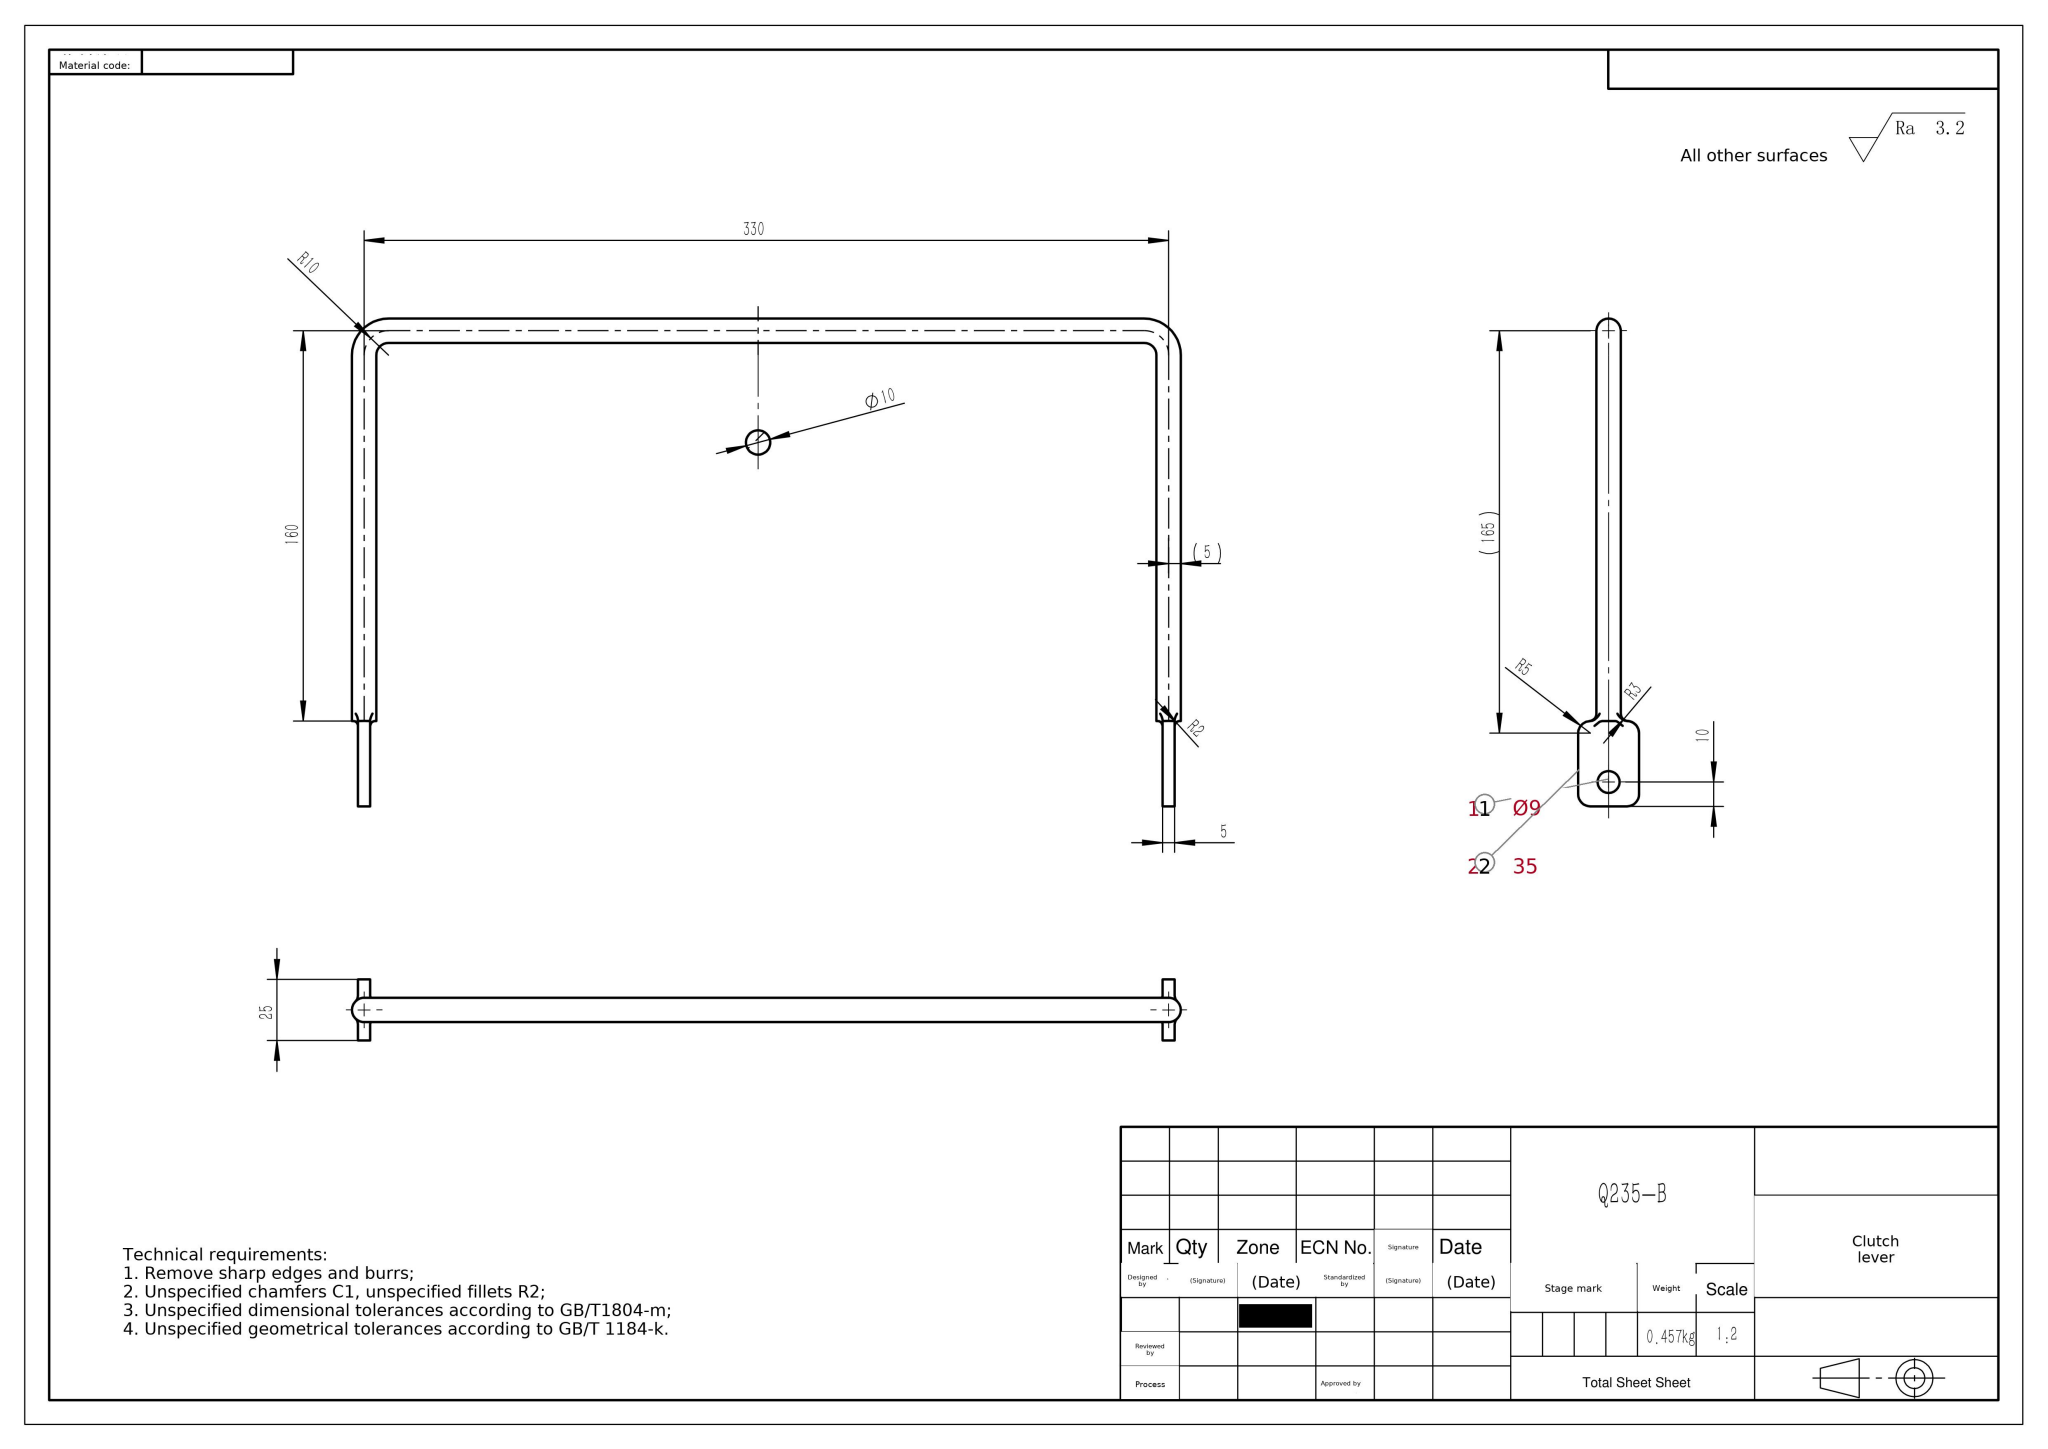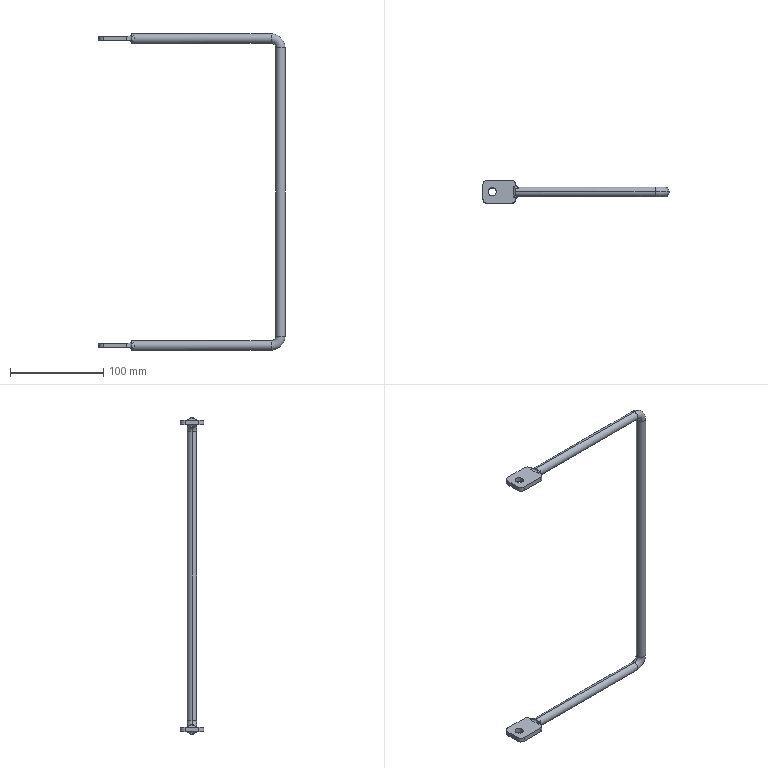Part | SolidWorks | mm | material Q235-B | 1 solid | 52 faces | box 200 x 25 x 340 mm | volume 58352 mm3 | cylinder 26 | plane 14 | torus 8 | spline 4 | commonest cylinder face diameters 10 x10 6 x8 9 x4 4 x4